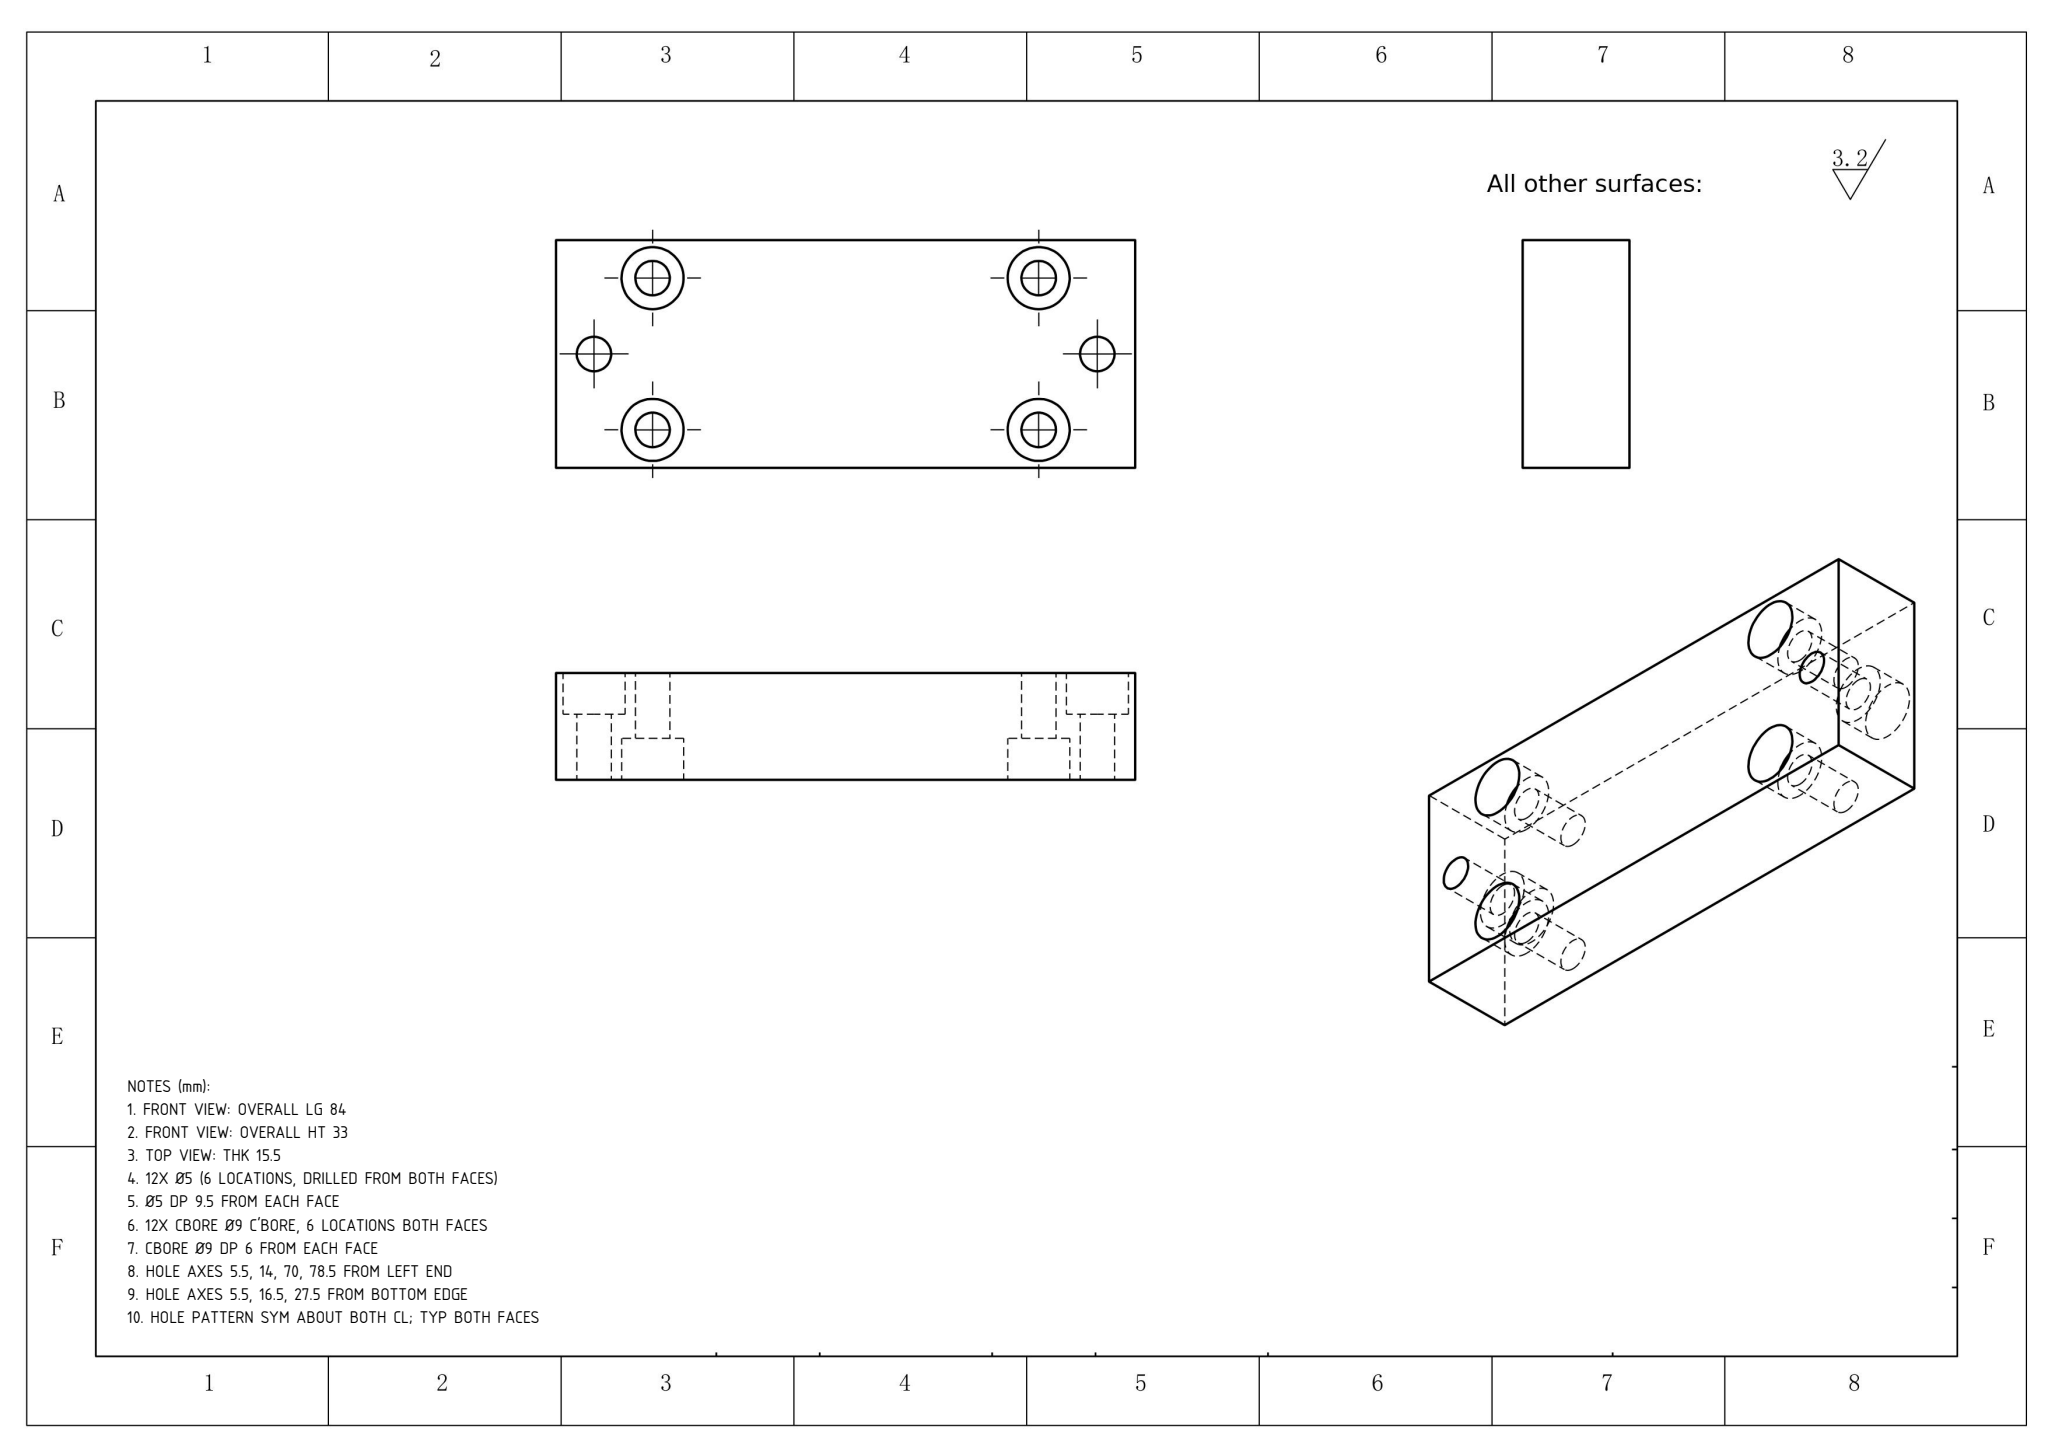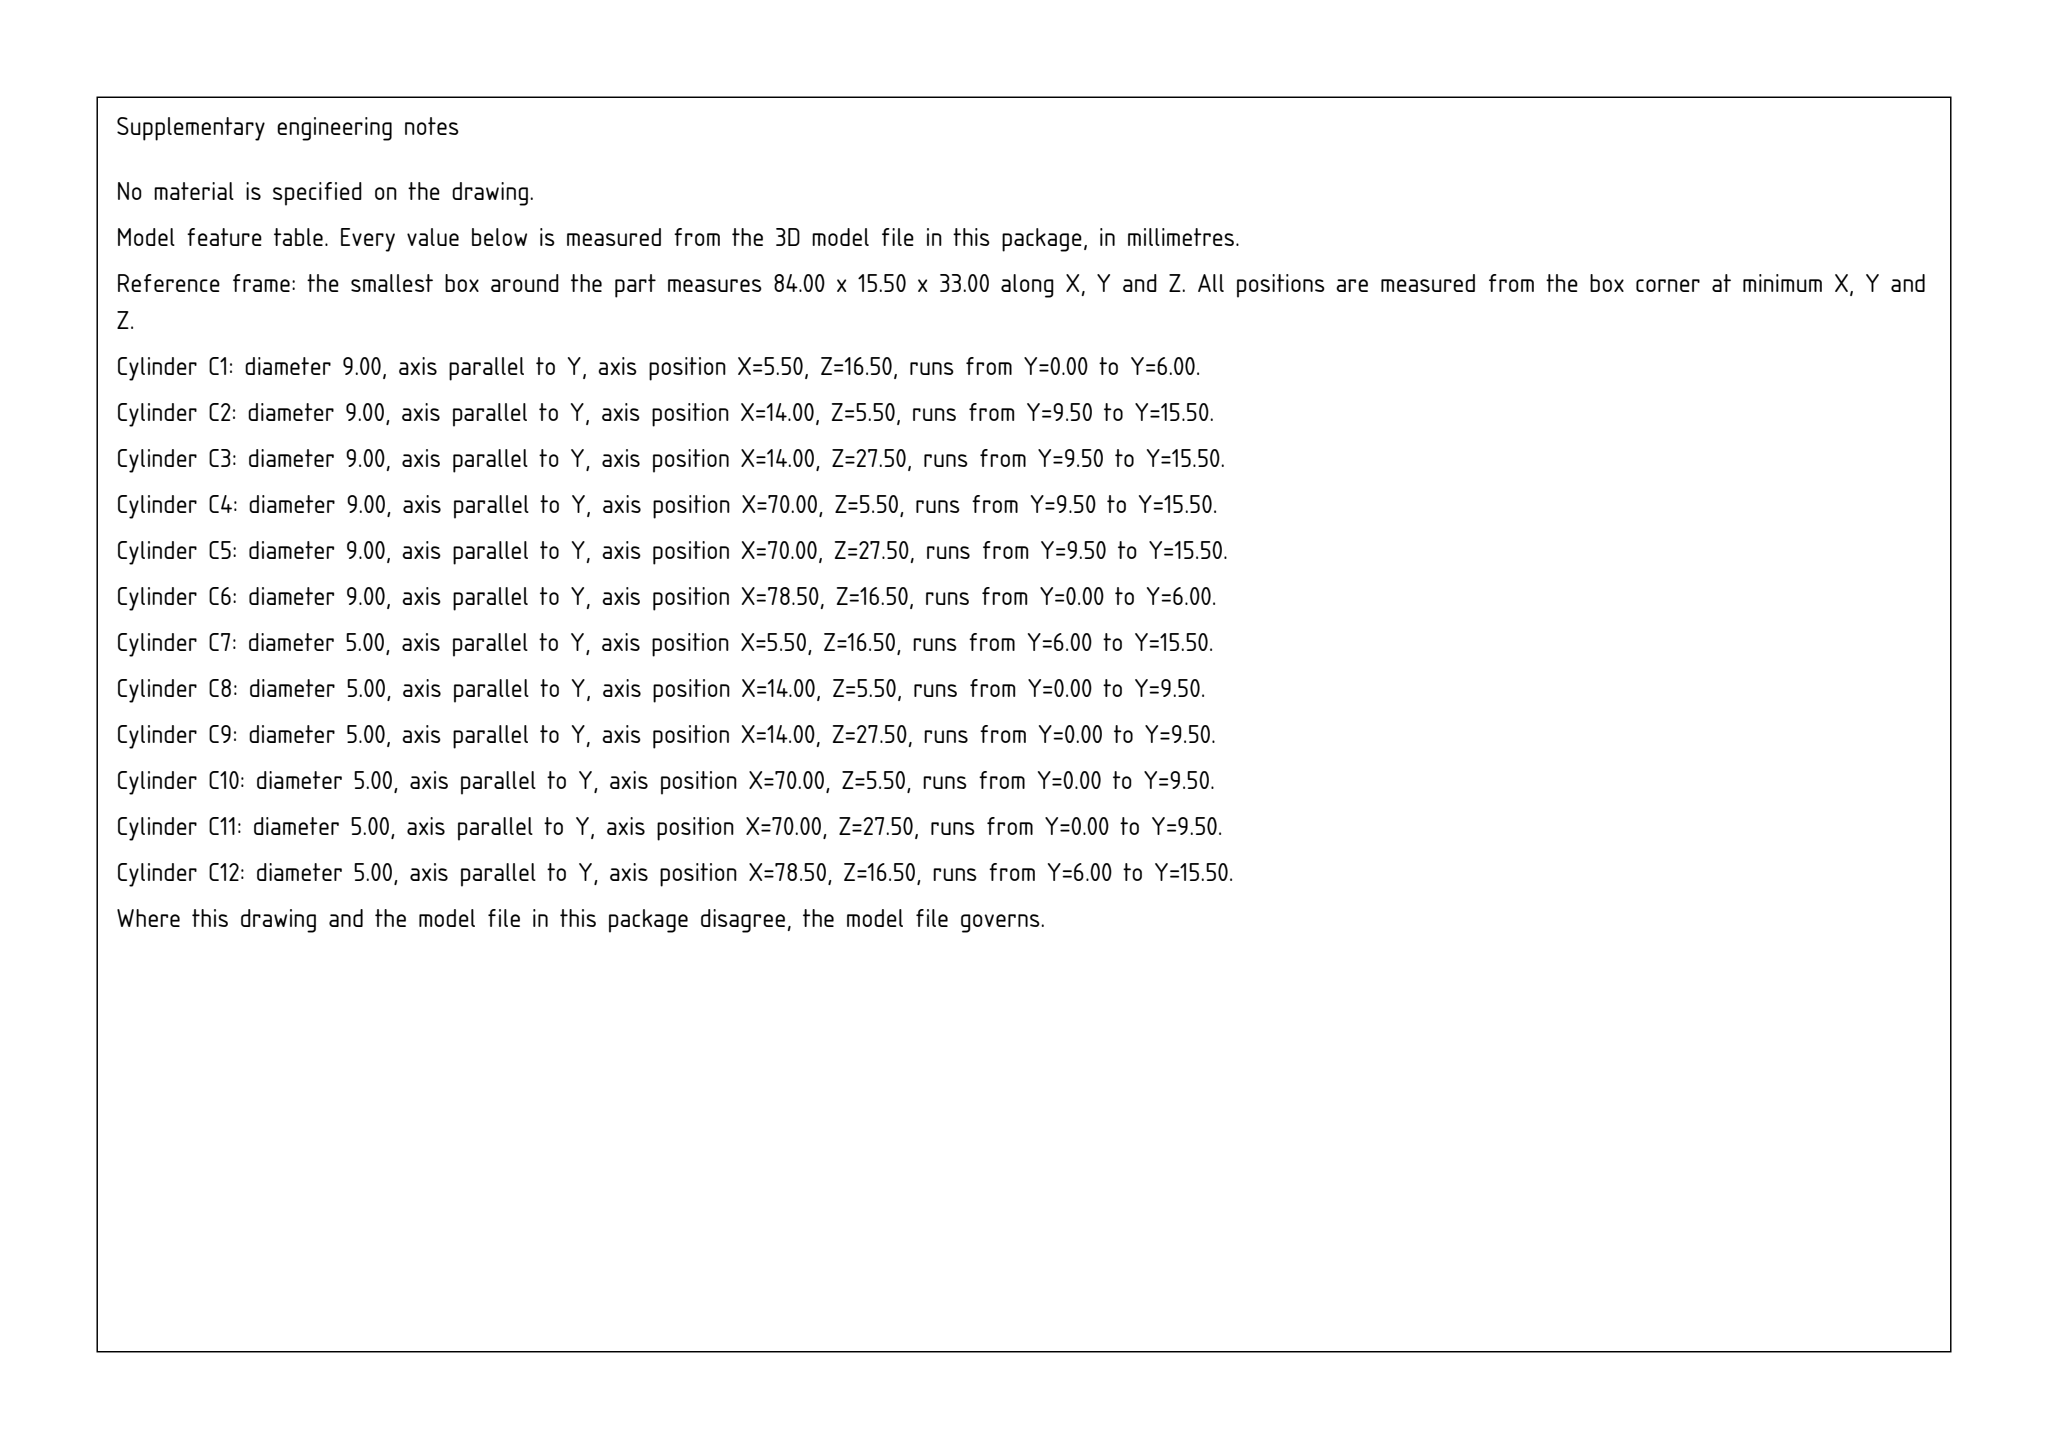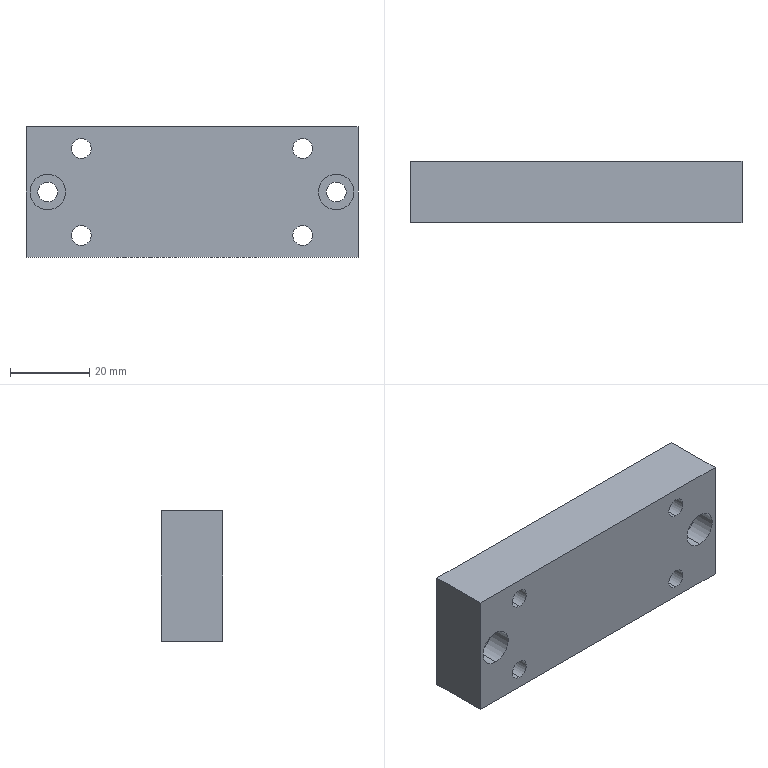Part | SolidWorks | mm | 1 solid | 36 faces | box 84 x 15.5 x 33 mm | volume 39557 mm3 | cylinder 24 | plane 12 | commonest cylinder face diameters 5 x12 9 x12
Drawing notes:
FRONT VIEW: OVERALL LG 84 | from the solid: bbox_xyz X = 84.0
FRONT VIEW: OVERALL HT 33 | from the solid: bbox_xyz Z = 33.0
TOP VIEW: THK 15.5 | from the solid: bbox_xyz Y = 15.5; planes y=0 and y=15.5
12X Ø5 (6 LOCATIONS, DRILLED FROM BOTH FACES) | from the solid: 12 cylinders dia 5.0, axis y, at 6 unique XZ positions
Ø5 DP 9.5 FROM EACH FACE | from the solid: dia 5.0 cylinders length 9.5 from y=0 and y=15.5
12X CBORE Ø9 C'BORE, 6 LOCATIONS BOTH FACES | from the solid: 12 cylinders dia 9.0, axis y, same 6 XZ positions
CBORE Ø9 DP 6 FROM EACH FACE | from the solid: dia 9.0 cylinders length 6.0; planes y=6.0 and y=9.5
HOLE AXES 5.5, 14, 70, 78.5 FROM LEFT END | from the solid: cylinder X positions 5.5, 14.0, 70.0, 78.5
HOLE AXES 5.5, 16.5, 27.5 FROM BOTTOM EDGE | from the solid: cylinder Z positions 5.5, 16.5, 27.5
HOLE PATTERN SYM ABOUT BOTH CL; TYP BOTH FACES | from the solid: X 5.5/78.5 & 14/70 and Z 5.5/27.5 sym about 42 and 16.5; 2 per hole
build123d program:
from build123d import *

# Parameters (mm, degrees)
SKETCH1_W                                            = 84
SKETCH1_H                                            = 33
EXTRUDE1_DEPTH                                       = 15.5
HOLE_SIZE_ACCORDING_TO_THE_TYPE_OF_HEXAG_D           = 5
HOLE_SIZE_ACCORDING_TO_THE_TYPE_OF_HEXAG_CBORE_D     = 9
HOLE_SIZE_ACCORDING_TO_THE_TYPE_OF_HEXAG_CBORE_DEPTH = 6
HOLE_SIZE_ACCORDING_TO_THE_TYPE_OF_H_2_D             = 5
HOLE_SIZE_ACCORDING_TO_THE_TYPE_OF_H_2_CBORE_D       = 9
HOLE_SIZE_ACCORDING_TO_THE_TYPE_OF_H_2_CBORE_DEPTH   = 6


with BuildPart() as part:
    # Sketch1 → Extrude1 (new body)
    with BuildSketch(Plane(origin=(0, 0, 0), x_dir=(1, 0, 0), z_dir=(0, 1, 0))):
        with Locations((-54.031, 34.233)):
            Rectangle(SKETCH1_W, SKETCH1_H)
    extrude(amount=EXTRUDE1_DEPTH)

    # Hole Size according to the type of hexag (through all)
    with Locations(Plane(origin=(-82.031, 15.5, -45.233), x_dir=(0, 0, 1), z_dir=(0, 1, 0))):
        with Locations((0, 0), (0, 56), (22, 0), (22, 56)):
            CounterBoreHole(HOLE_SIZE_ACCORDING_TO_THE_TYPE_OF_HEXAG_D / 2, HOLE_SIZE_ACCORDING_TO_THE_TYPE_OF_HEXAG_CBORE_D / 2, HOLE_SIZE_ACCORDING_TO_THE_TYPE_OF_HEXAG_CBORE_DEPTH)

    # Hole Size according to the type of h 2 (through all)
    with Locations(Plane(origin=(-90.531, 0, -34.233), x_dir=(0, 0, -1), z_dir=(0, -1, 0))):
        with Locations((0, 0), (0, 73)):
            CounterBoreHole(HOLE_SIZE_ACCORDING_TO_THE_TYPE_OF_H_2_D / 2, HOLE_SIZE_ACCORDING_TO_THE_TYPE_OF_H_2_CBORE_D / 2, HOLE_SIZE_ACCORDING_TO_THE_TYPE_OF_H_2_CBORE_DEPTH)


solid = part.part